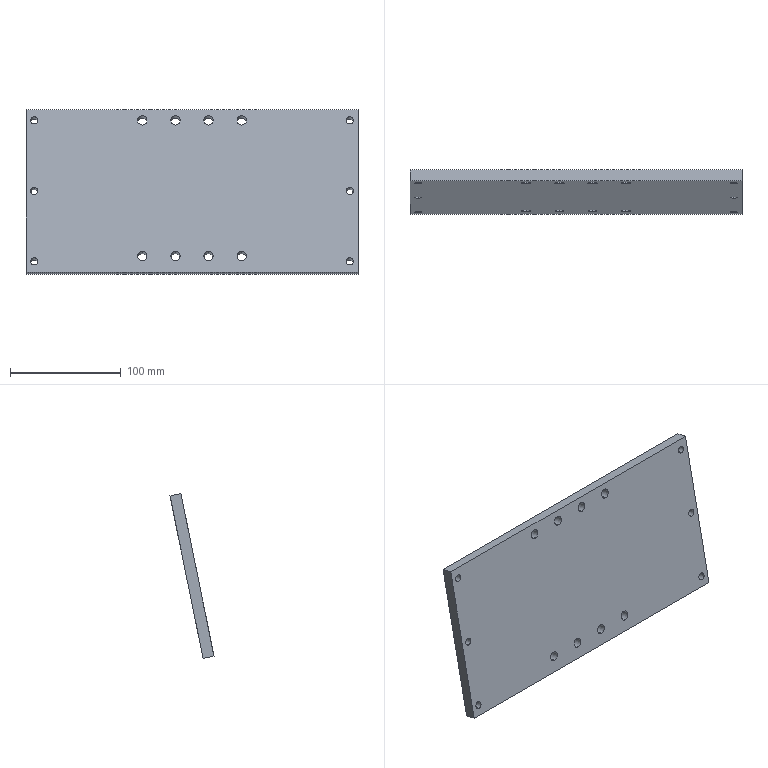Component | SolidWorks | JL001-04-01-002-1 | 1 solid | 34 faces | box 300 x 39.79 x 148.97 mm | volume 443469 mm3 | cylinder 28 | plane 6 | commonest cylinder face diameters 8.5 x16 6.5 x12
build123d program:
from build123d import *

# Parameters (mm, degrees)
SKETCH1_W                      = 300
SKETCH1_H                      = 150
BOSS_EXTRUDE1_DEPTH            = 10
F_6_5_6_5_DIAMETER_HOLE1_D     = 6.5
F_6_5_6_5_DIAMETER_HOLE1_DEPTH = 15
F_6_5_6_5_DIAMETER_HOLE1_TIP   = 1.953
F_8_5_8_5_DIAMETER_HOLE1_D     = 8.5
F_8_5_8_5_DIAMETER_HOLE1_DEPTH = 15
F_8_5_8_5_DIAMETER_HOLE1_TIP   = 2.554


with BuildPart() as part:
    # Sketch1 → Boss-Extrude1 (new body)
    with BuildSketch(Plane(origin=(0, 0, 0), x_dir=(1, 0, 0), z_dir=(0, 1, 0))):
        Rectangle(SKETCH1_W, SKETCH1_H)
    extrude(amount=BOSS_EXTRUDE1_DEPTH)

    # 6.5 _6.5_ Diameter Hole1
    with Locations(Plane(origin=(0, 10, 0), x_dir=(1, 0, 0), z_dir=(0, 1, 0))):
        with Locations((-142.5, 65), (-142.5, 0), (-142.5, -65), (142.5, 65), (142.5, 0), (142.5, -65)):
            Hole(F_6_5_6_5_DIAMETER_HOLE1_D / 2, depth=F_6_5_6_5_DIAMETER_HOLE1_DEPTH)
            with Locations((0, 0, -(F_6_5_6_5_DIAMETER_HOLE1_DEPTH + F_6_5_6_5_DIAMETER_HOLE1_TIP / 2))):  # 118° drill point
                Cone(0, F_6_5_6_5_DIAMETER_HOLE1_D / 2, F_6_5_6_5_DIAMETER_HOLE1_TIP, mode=Mode.SUBTRACT)

    # 8.5 _8.5_ Diameter Hole1
    with Locations(Plane(origin=(0, 10, 0), x_dir=(1, 0, 0), z_dir=(0, 1, 0))):
        with Locations((-45, 60), (-15, 60), (15, 60), (45, 60), (-45, -65), (-15, -65), (15, -65), (45, -65)):
            Hole(F_8_5_8_5_DIAMETER_HOLE1_D / 2, depth=F_8_5_8_5_DIAMETER_HOLE1_DEPTH)
            with Locations((0, 0, -(F_8_5_8_5_DIAMETER_HOLE1_DEPTH + F_8_5_8_5_DIAMETER_HOLE1_TIP / 2))):  # 118° drill point
                Cone(0, F_8_5_8_5_DIAMETER_HOLE1_D / 2, F_8_5_8_5_DIAMETER_HOLE1_TIP, mode=Mode.SUBTRACT)


solid = part.part

# Placed as in the assembly
solid = solid.moved(Location((0, 119.997, 73.485), (-11.535, 0, 0)))